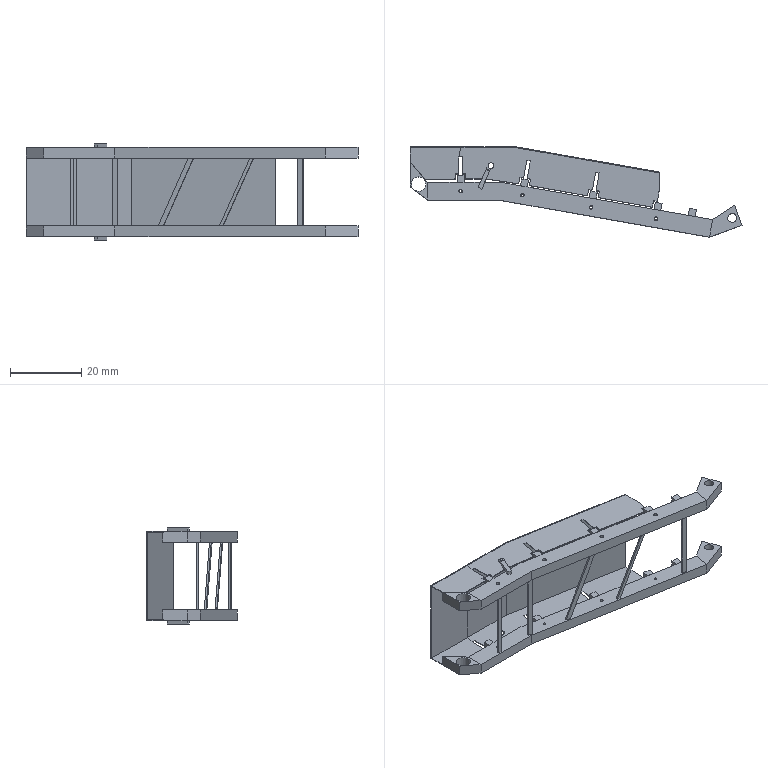Component | NX | HH | 29 solids | 352 faces | volume 3616 mm3 | plane 305 | cylinder 41 | sphere 4 | spline 2 | commonest cylinder face diameters 0.086 x14 0.8 x8 1 x8 2.493 x2 1.684 x2 4 x2 0.628 x2 0.394 x2